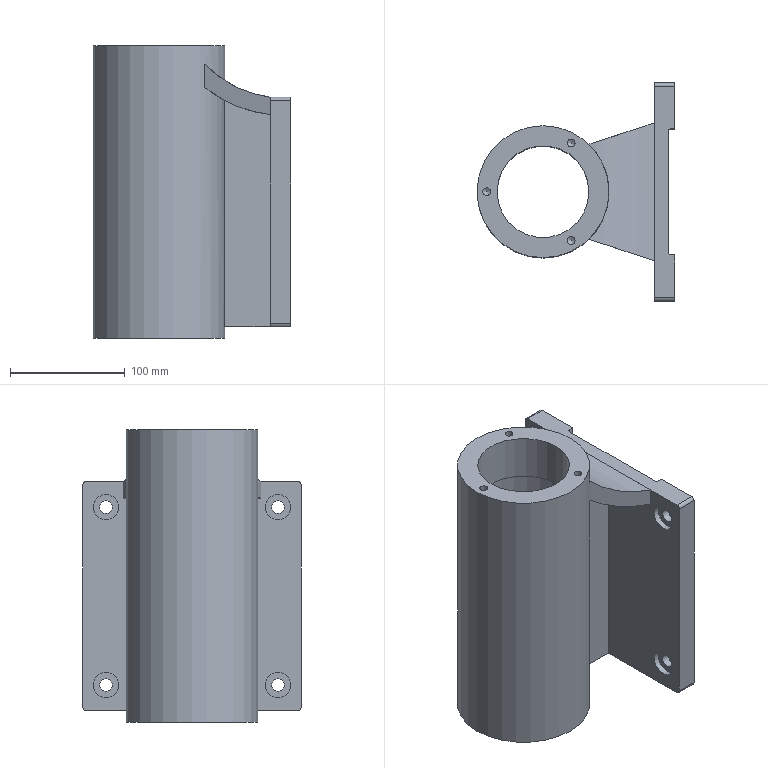Component | NX | GAS_ENGINE_BRACKET | 2 solids | 57 faces | volume 1705293 mm3 | cylinder 27 | plane 24 | cone 6 | commonest cylinder face diameters 6.8 x6 6 x6 11 x4 22 x4 220 x2 80 x2 190 x1 115 x1